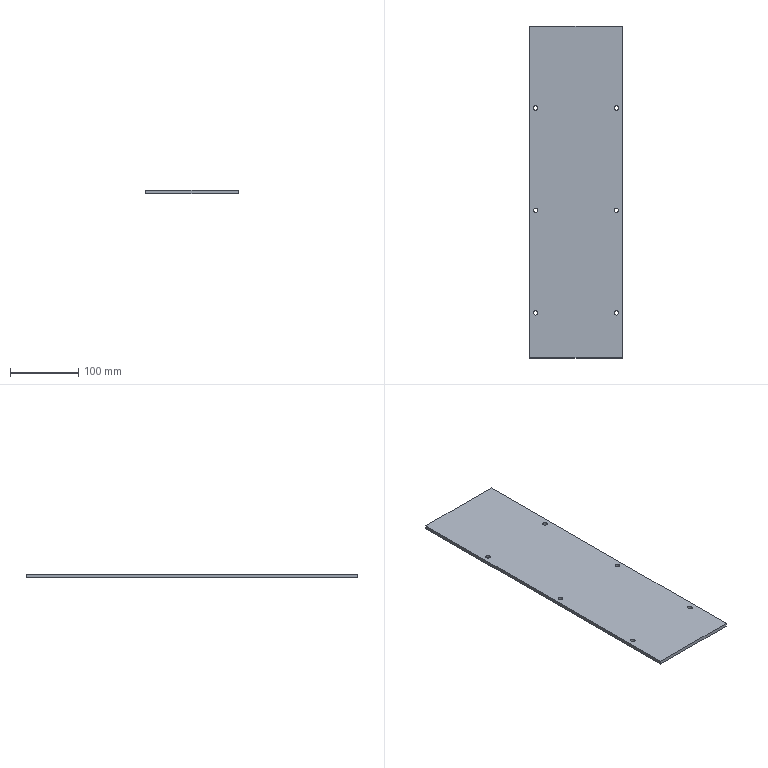Component | SolidWorks | ZL-11-03LargeUprightPlate-3 | 1 solid | 18 faces | box 136 x 486 x 5 mm | volume 329485 mm3 | cylinder 12 | plane 6 | commonest cylinder face diameters 6.5 x12
build123d program:
from build123d import *

# Parameters (mm, degrees)
SKETCH1_W                  = 136
SKETCH1_H                  = 486
EXTRUDE1_DEPTH             = 5
F_6_5_6_5_DIAMETER_HOLE1_D = 6.5
LPATTERN1_COUNT            = 2
LPATTERN1_PITCH            = 118
LPATTERN1_COUNT_DIR2       = 3
LPATTERN1_PITCH_DIR2       = 150


with BuildPart() as part:
    # Sketch1 → Extrude1 (new body)
    with BuildSketch(Plane.XY):
        Rectangle(SKETCH1_W, SKETCH1_H)
    extrude(amount=EXTRUDE1_DEPTH)

    # 6.5 _6.5_ Diameter Hole1 (through all)
    with Locations(Plane(origin=(-59, 123, 5), x_dir=(1, 0, 0), z_dir=(0, 0, 1))):
        with Locations((0, 0)):
            f_6_5_6_5_diameter_hole1 = Hole(F_6_5_6_5_DIAMETER_HOLE1_D / 2)

    # LPattern1: 6.5 _6.5_ Diameter Hole1 2 × 3
    with Locations(*[(i * LPATTERN1_PITCH, -j * LPATTERN1_PITCH_DIR2, 0) for i in range(LPATTERN1_COUNT) for j in range(LPATTERN1_COUNT_DIR2) if (i, j) != (0, 0)]):
        add(f_6_5_6_5_diameter_hole1, mode=Mode.SUBTRACT)


solid = part.part

# Placed as in the assembly
solid = solid.moved(Location((125.552, 281.22, 60.5), (0, 0, 0)))
STEP:
#1=CARTESIAN_POINT('',(7.138,4.103,2.382));
#2=VERTEX_POINT('',#1);
#3=CARTESIAN_POINT('',(7.394,4.103,2.382));
#4=VERTEX_POINT('',#3);
#5=CARTESIAN_POINT('',(7.266,4.103,2.382));
#6=DIRECTION('',(0.,0.,1.));
#7=DIRECTION('',(1.,0.,0.));
#8=AXIS2_PLACEMENT_3D('',#5,#6,#7);
#9=CIRCLE('',#8,0.128);
#10=EDGE_CURVE('',#2,#4,#9,.T.);
#11=ORIENTED_EDGE('',*,*,#10,.F.);
#12=CARTESIAN_POINT('',(7.138,4.103,2.579));
#13=VERTEX_POINT('',#12);
#14=CARTESIAN_POINT('',(7.138,4.103,2.579));
#15=DIRECTION('',(0.,0.,1.));
#16=VECTOR('',#15,39.37);
#17=LINE('',#14,#16);
#18=EDGE_CURVE('',#2,#13,#17,.T.);
#19=ORIENTED_EDGE('',*,*,#18,.T.);
#20=CARTESIAN_POINT('',(7.394,4.103,2.579));
#21=VERTEX_POINT('',#20);
#22=CARTESIAN_POINT('',(7.266,4.103,2.579));
#23=DIRECTION('',(0.,0.,1.));
#24=DIRECTION('',(1.,0.,0.));
#25=AXIS2_PLACEMENT_3D('',#22,#23,#24);
#26=CIRCLE('',#25,0.128);
#27=EDGE_CURVE('',#13,#21,#26,.T.);
#28=ORIENTED_EDGE('',*,*,#27,.T.);
#29=CARTESIAN_POINT('',(7.394,4.103,2.579));
#30=DIRECTION('',(0.,0.,1.));
#31=VECTOR('',#30,39.37);
#32=LINE('',#29,#31);
#33=EDGE_CURVE('',#4,#21,#32,.T.);
#34=ORIENTED_EDGE('',*,*,#33,.F.);
#35=EDGE_LOOP('',(#11,#19,#28,#34));
#36=FACE_OUTER_BOUND('',#35,.T.);
#37=CARTESIAN_POINT('',(7.266,4.103,2.579));
#38=DIRECTION('',(0.,0.,1.));
#39=DIRECTION('',(1.,0.,0.));
#40=AXIS2_PLACEMENT_3D('',#37,#38,#39);
#41=CYLINDRICAL_SURFACE('',#40,0.128);
#42=ADVANCED_FACE('',(#36),#41,.F.);
#43=CARTESIAN_POINT('',(7.138,10.009,2.382));
#44=VERTEX_POINT('',#43);
#45=CARTESIAN_POINT('',(7.394,10.009,2.382));
#46=VERTEX_POINT('',#45);
#47=CARTESIAN_POINT('',(7.266,10.009,2.382));
#48=DIRECTION('',(0.,0.,1.));
#49=DIRECTION('',(1.,0.,0.));
#50=AXIS2_PLACEMENT_3D('',#47,#48,#49);
#51=CIRCLE('',#50,0.128);
#52=EDGE_CURVE('',#44,#46,#51,.T.);
#53=ORIENTED_EDGE('',*,*,#52,.F.);
#54=CARTESIAN_POINT('',(7.138,10.009,2.579));
#55=VERTEX_POINT('',#54);
#56=CARTESIAN_POINT('',(7.138,10.009,2.579));
#57=DIRECTION('',(0.,0.,1.));
#58=VECTOR('',#57,39.37);
#59=LINE('',#56,#58);
#60=EDGE_CURVE('',#44,#55,#59,.T.);
#61=ORIENTED_EDGE('',*,*,#60,.T.);
#62=CARTESIAN_POINT('',(7.394,10.009,2.579));
#63=VERTEX_POINT('',#62);
#64=CARTESIAN_POINT('',(7.266,10.009,2.579));
#65=DIRECTION('',(0.,0.,1.));
#66=DIRECTION('',(1.,0.,0.));
#67=AXIS2_PLACEMENT_3D('',#64,#65,#66);
#68=CIRCLE('',#67,0.128);
#69=EDGE_CURVE('',#55,#63,#68,.T.);
#70=ORIENTED_EDGE('',*,*,#69,.T.);
#71=CARTESIAN_POINT('',(7.394,10.009,2.579));
#72=DIRECTION('',(0.,0.,1.));
#73=VECTOR('',#72,39.37);
#74=LINE('',#71,#73);
#75=EDGE_CURVE('',#46,#63,#74,.T.);
#76=ORIENTED_EDGE('',*,*,#75,.F.);
#77=EDGE_LOOP('',(#53,#61,#70,#76));
#78=FACE_OUTER_BOUND('',#77,.T.);
#79=CARTESIAN_POINT('',(7.266,10.009,2.579));
#80=DIRECTION('',(0.,0.,1.));
#81=DIRECTION('',(1.,0.,0.));
#82=AXIS2_PLACEMENT_3D('',#79,#80,#81);
#83=CYLINDRICAL_SURFACE('',#82,0.128);
#84=ADVANCED_FACE('',(#78),#83,.F.);
#85=CARTESIAN_POINT('',(7.138,15.914,2.382));
#86=VERTEX_POINT('',#85);
#87=CARTESIAN_POINT('',(7.394,15.914,2.382));
#88=VERTEX_POINT('',#87);
#89=CARTESIAN_POINT('',(7.266,15.914,2.382));
#90=DIRECTION('',(0.,0.,1.));
#91=DIRECTION('',(1.,0.,0.));
#92=AXIS2_PLACEMENT_3D('',#89,#90,#91);
#93=CIRCLE('',#92,0.128);
#94=EDGE_CURVE('',#86,#88,#93,.T.);
#95=ORIENTED_EDGE('',*,*,#94,.F.);
#96=CARTESIAN_POINT('',(7.138,15.914,2.579));
#97=VERTEX_POINT('',#96);
#98=CARTESIAN_POINT('',(7.138,15.914,2.579));
#99=DIRECTION('',(0.,0.,1.));
#100=VECTOR('',#99,39.37);
#101=LINE('',#98,#100);
#102=EDGE_CURVE('',#86,#97,#101,.T.);
#103=ORIENTED_EDGE('',*,*,#102,.T.);
#104=CARTESIAN_POINT('',(7.394,15.914,2.579));
#105=VERTEX_POINT('',#104);
#106=CARTESIAN_POINT('',(7.266,15.914,2.579));
#107=DIRECTION('',(0.,0.,1.));
#108=DIRECTION('',(1.,0.,0.));
#109=AXIS2_PLACEMENT_3D('',#106,#107,#108);
#110=CIRCLE('',#109,0.128);
#111=EDGE_CURVE('',#97,#105,#110,.T.);
#112=ORIENTED_EDGE('',*,*,#111,.T.);
#113=CARTESIAN_POINT('',(7.394,15.914,2.579));
#114=DIRECTION('',(0.,0.,1.));
#115=VECTOR('',#114,39.37);
#116=LINE('',#113,#115);
#117=EDGE_CURVE('',#88,#105,#116,.T.);
#118=ORIENTED_EDGE('',*,*,#117,.F.);
#119=EDGE_LOOP('',(#95,#103,#112,#118));
#120=FACE_OUTER_BOUND('',#119,.T.);
#121=CARTESIAN_POINT('',(7.266,15.914,2.579));
#122=DIRECTION('',(0.,0.,1.));
#123=DIRECTION('',(1.,0.,0.));
#124=AXIS2_PLACEMENT_3D('',#121,#122,#123);
#125=CYLINDRICAL_SURFACE('',#124,0.128);
#126=ADVANCED_FACE('',(#120),#125,.F.);
#127=CARTESIAN_POINT('',(2.492,4.103,2.382));
#128=VERTEX_POINT('',#127);
#129=CARTESIAN_POINT('',(2.748,4.103,2.382));
#130=VERTEX_POINT('',#129);
#131=CARTESIAN_POINT('',(2.62,4.103,2.382));
#132=DIRECTION('',(0.,0.,1.));
#133=DIRECTION('',(1.,0.,0.));
#134=AXIS2_PLACEMENT_3D('',#131,#132,#133);
#135=CIRCLE('',#134,0.128);
#136=EDGE_CURVE('',#128,#130,#135,.T.);
#137=ORIENTED_EDGE('',*,*,#136,.F.);
#138=CARTESIAN_POINT('',(2.492,4.103,2.579));
#139=VERTEX_POINT('',#138);
#140=CARTESIAN_POINT('',(2.492,4.103,2.579));
#141=DIRECTION('',(0.,0.,1.));
#142=VECTOR('',#141,39.37);
#143=LINE('',#140,#142);
#144=EDGE_CURVE('',#128,#139,#143,.T.);
#145=ORIENTED_EDGE('',*,*,#144,.T.);
#146=CARTESIAN_POINT('',(2.748,4.103,2.579));
#147=VERTEX_POINT('',#146);
#148=CARTESIAN_POINT('',(2.62,4.103,2.579));
#149=DIRECTION('',(0.,0.,1.));
#150=DIRECTION('',(1.,0.,0.));
#151=AXIS2_PLACEMENT_3D('',#148,#149,#150);
#152=CIRCLE('',#151,0.128);
#153=EDGE_CURVE('',#139,#147,#152,.T.);
#154=ORIENTED_EDGE('',*,*,#153,.T.);
#155=CARTESIAN_POINT('',(2.748,4.103,2.579));
#156=DIRECTION('',(0.,0.,1.));
#157=VECTOR('',#156,39.37);
#158=LINE('',#155,#157);
#159=EDGE_CURVE('',#130,#147,#158,.T.);
#160=ORIENTED_EDGE('',*,*,#159,.F.);
#161=EDGE_LOOP('',(#137,#145,#154,#160));
#162=FACE_OUTER_BOUND('',#161,.T.);
#163=CARTESIAN_POINT('',(2.62,4.103,2.579));
#164=DIRECTION('',(0.,0.,1.));
#165=DIRECTION('',(1.,0.,0.));
#166=AXIS2_PLACEMENT_3D('',#163,#164,#165);
#167=CYLINDRICAL_SURFACE('',#166,0.128);
#168=ADVANCED_FACE('',(#162),#167,.F.);
#169=CARTESIAN_POINT('',(2.492,10.009,2.382));
#170=VERTEX_POINT('',#169);
#171=CARTESIAN_POINT('',(2.748,10.009,2.382));
#172=VERTEX_POINT('',#171);
#173=CARTESIAN_POINT('',(2.62,10.009,2.382));
#174=DIRECTION('',(0.,0.,1.));
#175=DIRECTION('',(1.,0.,0.));
#176=AXIS2_PLACEMENT_3D('',#173,#174,#175);
#177=CIRCLE('',#176,0.128);
#178=EDGE_CURVE('',#170,#172,#177,.T.);
#179=ORIENTED_EDGE('',*,*,#178,.F.);
#180=CARTESIAN_POINT('',(2.492,10.009,2.579));
#181=VERTEX_POINT('',#180);
#182=CARTESIAN_POINT('',(2.492,10.009,2.579));
#183=DIRECTION('',(0.,0.,1.));
#184=VECTOR('',#183,39.37);
#185=LINE('',#182,#184);
#186=EDGE_CURVE('',#170,#181,#185,.T.);
#187=ORIENTED_EDGE('',*,*,#186,.T.);
#188=CARTESIAN_POINT('',(2.748,10.009,2.579));
#189=VERTEX_POINT('',#188);
#190=CARTESIAN_POINT('',(2.62,10.009,2.579));
#191=DIRECTION('',(0.,0.,1.));
#192=DIRECTION('',(1.,0.,0.));
#193=AXIS2_PLACEMENT_3D('',#190,#191,#192);
#194=CIRCLE('',#193,0.128);
#195=EDGE_CURVE('',#181,#189,#194,.T.);
#196=ORIENTED_EDGE('',*,*,#195,.T.);
#197=CARTESIAN_POINT('',(2.748,10.009,2.579));
#198=DIRECTION('',(0.,0.,1.));
#199=VECTOR('',#198,39.37);
#200=LINE('',#197,#199);
#201=EDGE_CURVE('',#172,#189,#200,.T.);
#202=ORIENTED_EDGE('',*,*,#201,.F.);
#203=EDGE_LOOP('',(#179,#187,#196,#202));
#204=FACE_OUTER_BOUND('',#203,.T.);
#205=CARTESIAN_POINT('',(2.62,10.009,2.579));
#206=DIRECTION('',(0.,0.,1.));
#207=DIRECTION('',(1.,0.,0.));
#208=AXIS2_PLACEMENT_3D('',#205,#206,#207);
#209=CYLINDRICAL_SURFACE('',#208,0.128);
#210=ADVANCED_FACE('',(#204),#209,.F.);
#211=CARTESIAN_POINT('',(2.492,15.914,2.382));
#212=VERTEX_POINT('',#211);
#213=CARTESIAN_POINT('',(2.748,15.914,2.382));
#214=VERTEX_POINT('',#213);
#215=CARTESIAN_POINT('',(2.62,15.914,2.382));
#216=DIRECTION('',(0.,0.,1.));
#217=DIRECTION('',(1.,0.,0.));
#218=AXIS2_PLACEMENT_3D('',#215,#216,#217);
#219=CIRCLE('',#218,0.128);
#220=EDGE_CURVE('',#212,#214,#219,.T.);
#221=ORIENTED_EDGE('',*,*,#220,.F.);
#222=CARTESIAN_POINT('',(2.492,15.914,2.579));
#223=VERTEX_POINT('',#222);
#224=CARTESIAN_POINT('',(2.492,15.914,2.579));
#225=DIRECTION('',(0.,0.,1.));
#226=VECTOR('',#225,39.37);
#227=LINE('',#224,#226);
#228=EDGE_CURVE('',#212,#223,#227,.T.);
#229=ORIENTED_EDGE('',*,*,#228,.T.);
#230=CARTESIAN_POINT('',(2.748,15.914,2.579));
#231=VERTEX_POINT('',#230);
#232=CARTESIAN_POINT('',(2.62,15.914,2.579));
#233=DIRECTION('',(0.,0.,1.));
#234=DIRECTION('',(1.,0.,0.));
#235=AXIS2_PLACEMENT_3D('',#232,#233,#234);
#236=CIRCLE('',#235,0.128);
#237=EDGE_CURVE('',#223,#231,#236,.T.);
#238=ORIENTED_EDGE('',*,*,#237,.T.);
#239=CARTESIAN_POINT('',(2.748,15.914,2.579));
#240=DIRECTION('',(0.,0.,1.));
#241=VECTOR('',#240,39.37);
#242=LINE('',#239,#241);
#243=EDGE_CURVE('',#214,#231,#242,.T.);
#244=ORIENTED_EDGE('',*,*,#243,.F.);
#245=EDGE_LOOP('',(#221,#229,#238,#244));
#246=FACE_OUTER_BOUND('',#245,.T.);
#247=CARTESIAN_POINT('',(2.62,15.914,2.579));
#248=DIRECTION('',(0.,0.,1.));
#249=DIRECTION('',(1.,0.,0.));
#250=AXIS2_PLACEMENT_3D('',#247,#248,#249);
#251=CYLINDRICAL_SURFACE('',#250,0.128);
#252=ADVANCED_FACE('',(#246),#251,.F.);
#253=CARTESIAN_POINT('',(2.266,20.639,2.382));
#254=VERTEX_POINT('',#253);
#255=CARTESIAN_POINT('',(2.266,1.505,2.382));
#256=VERTEX_POINT('',#255);
#257=CARTESIAN_POINT('',(2.266,20.639,2.382));
#258=DIRECTION('',(0.,-1.,0.));
#259=VECTOR('',#258,39.37);
#260=LINE('',#257,#259);
#261=EDGE_CURVE('',#254,#256,#260,.T.);
#262=ORIENTED_EDGE('',*,*,#261,.T.);
#263=CARTESIAN_POINT('',(2.266,1.505,2.579));
#264=VERTEX_POINT('',#263);
#265=CARTESIAN_POINT('',(2.266,1.505,2.579));
#266=DIRECTION('',(0.,0.,-1.));
#267=VECTOR('',#266,39.37);
#268=LINE('',#265,#267);
#269=EDGE_CURVE('',#264,#256,#268,.T.);
#270=ORIENTED_EDGE('',*,*,#269,.F.);
#271=CARTESIAN_POINT('',(2.266,20.639,2.579));
#272=VERTEX_POINT('',#271);
#273=CARTESIAN_POINT('',(2.266,20.639,2.579));
#274=DIRECTION('',(0.,-1.,0.));
#275=VECTOR('',#274,39.37);
#276=LINE('',#273,#275);
#277=EDGE_CURVE('',#272,#264,#276,.T.);
#278=ORIENTED_EDGE('',*,*,#277,.F.);
#279=CARTESIAN_POINT('',(2.266,20.639,2.579));
#280=DIRECTION('',(0.,0.,-1.));
#281=VECTOR('',#280,39.37);
#282=LINE('',#279,#281);
#283=EDGE_CURVE('',#272,#254,#282,.T.);
#284=ORIENTED_EDGE('',*,*,#283,.T.);
#285=EDGE_LOOP('',(#262,#270,#278,#284));
#286=FACE_OUTER_BOUND('',#285,.T.);
#287=CARTESIAN_POINT('',(2.266,20.639,2.579));
#288=DIRECTION('',(1.,0.,0.));
#289=DIRECTION('',(-0.,1.,0.));
#290=AXIS2_PLACEMENT_3D('',#287,#288,#289);
#291=PLANE('',#290);
#292=ADVANCED_FACE('',(#286),#291,.F.);
#293=CARTESIAN_POINT('',(7.62,1.505,2.382));
#294=VERTEX_POINT('',#293);
#295=CARTESIAN_POINT('',(2.266,1.505,2.382));
#296=DIRECTION('',(1.,0.,0.));
#297=VECTOR('',#296,39.37);
#298=LINE('',#295,#297);
#299=EDGE_CURVE('',#256,#294,#298,.T.);
#300=ORIENTED_EDGE('',*,*,#299,.T.);
#301=CARTESIAN_POINT('',(7.62,1.505,2.579));
#302=VERTEX_POINT('',#301);
#303=CARTESIAN_POINT('',(7.62,1.505,2.579));
#304=DIRECTION('',(0.,0.,-1.));
#305=VECTOR('',#304,39.37);
#306=LINE('',#303,#305);
#307=EDGE_CURVE('',#302,#294,#306,.T.);
#308=ORIENTED_EDGE('',*,*,#307,.F.);
#309=CARTESIAN_POINT('',(2.266,1.505,2.579));
#310=DIRECTION('',(1.,0.,0.));
#311=VECTOR('',#310,39.37);
#312=LINE('',#309,#311);
#313=EDGE_CURVE('',#264,#302,#312,.T.);
#314=ORIENTED_EDGE('',*,*,#313,.F.);
#315=ORIENTED_EDGE('',*,*,#269,.T.);
#316=EDGE_LOOP('',(#300,#308,#314,#315));
#317=FACE_OUTER_BOUND('',#316,.T.);
#318=CARTESIAN_POINT('',(2.266,1.505,2.579));
#319=DIRECTION('',(-0.,1.,0.));
#320=DIRECTION('',(-1.,-0.,0.));
#321=AXIS2_PLACEMENT_3D('',#318,#319,#320);
#322=PLANE('',#321);
#323=ADVANCED_FACE('',(#317),#322,.F.);
#324=CARTESIAN_POINT('',(7.62,20.639,2.382));
#325=VERTEX_POINT('',#324);
#326=CARTESIAN_POINT('',(7.62,20.639,2.382));
#327=DIRECTION('',(-0.,1.,0.));
#328=VECTOR('',#327,39.37);
#329=LINE('',#326,#328);
#330=EDGE_CURVE('',#294,#325,#329,.T.);
#331=ORIENTED_EDGE('',*,*,#330,.T.);
#332=CARTESIAN_POINT('',(7.62,20.639,2.579));
#333=VERTEX_POINT('',#332);
#334=CARTESIAN_POINT('',(7.62,20.639,2.579));
#335=DIRECTION('',(0.,0.,-1.));
#336=VECTOR('',#335,39.37);
#337=LINE('',#334,#336);
#338=EDGE_CURVE('',#333,#325,#337,.T.);
#339=ORIENTED_EDGE('',*,*,#338,.F.);
#340=CARTESIAN_POINT('',(7.62,20.639,2.579));
#341=DIRECTION('',(-0.,1.,0.));
#342=VECTOR('',#341,39.37);
#343=LINE('',#340,#342);
#344=EDGE_CURVE('',#302,#333,#343,.T.);
#345=ORIENTED_EDGE('',*,*,#344,.F.);
#346=ORIENTED_EDGE('',*,*,#307,.T.);
#347=EDGE_LOOP('',(#331,#339,#345,#346));
#348=FACE_OUTER_BOUND('',#347,.T.);
#349=CARTESIAN_POINT('',(7.62,20.639,2.579));
#350=DIRECTION('',(-1.,-0.,0.));
#351=DIRECTION('',(0.,-1.,0.));
#352=AXIS2_PLACEMENT_3D('',#349,#350,#351);
#353=PLANE('',#352);
#354=ADVANCED_FACE('',(#348),#353,.F.);
#355=CARTESIAN_POINT('',(2.266,20.639,2.382));
#356=DIRECTION('',(-1.,-0.,0.));
#357=VECTOR('',#356,39.37);
#358=LINE('',#355,#357);
#359=EDGE_CURVE('',#325,#254,#358,.T.);
#360=ORIENTED_EDGE('',*,*,#359,.T.);
#361=ORIENTED_EDGE('',*,*,#283,.F.);
#362=CARTESIAN_POINT('',(2.266,20.639,2.579));
#363=DIRECTION('',(-1.,-0.,0.));
#364=VECTOR('',#363,39.37);
#365=LINE('',#362,#364);
#366=EDGE_CURVE('',#333,#272,#365,.T.);
#367=ORIENTED_EDGE('',*,*,#366,.F.);
#368=ORIENTED_EDGE('',*,*,#338,.T.);
#369=EDGE_LOOP('',(#360,#361,#367,#368));
#370=FACE_OUTER_BOUND('',#369,.T.);
#371=CARTESIAN_POINT('',(2.266,20.639,2.579));
#372=DIRECTION('',(0.,-1.,0.));
#373=DIRECTION('',(1.,0.,0.));
#374=AXIS2_PLACEMENT_3D('',#371,#372,#373);
#375=PLANE('',#374);
#376=ADVANCED_FACE('',(#370),#375,.F.);
#377=CARTESIAN_POINT('',(7.266,4.103,2.579));
#378=DIRECTION('',(0.,0.,1.));
#379=DIRECTION('',(1.,0.,0.));
#380=AXIS2_PLACEMENT_3D('',#377,#378,#379);
#381=CIRCLE('',#380,0.128);
#382=EDGE_CURVE('',#21,#13,#381,.T.);
#383=ORIENTED_EDGE('',*,*,#382,.F.);
#384=ORIENTED_EDGE('',*,*,#27,.F.);
#385=EDGE_LOOP('',(#383,#384));
#386=FACE_BOUND('',#385,.T.);
#387=CARTESIAN_POINT('',(7.266,10.009,2.579));
#388=DIRECTION('',(0.,0.,1.));
#389=DIRECTION('',(1.,0.,0.));
#390=AXIS2_PLACEMENT_3D('',#387,#388,#389);
#391=CIRCLE('',#390,0.128);
#392=EDGE_CURVE('',#63,#55,#391,.T.);
#393=ORIENTED_EDGE('',*,*,#392,.F.);
#394=ORIENTED_EDGE('',*,*,#69,.F.);
#395=EDGE_LOOP('',(#393,#394));
#396=FACE_BOUND('',#395,.T.);
#397=CARTESIAN_POINT('',(7.266,15.914,2.579));
#398=DIRECTION('',(0.,0.,1.));
#399=DIRECTION('',(1.,0.,0.));
#400=AXIS2_PLACEMENT_3D('',#397,#398,#399);
#401=CIRCLE('',#400,0.128);
#402=EDGE_CURVE('',#105,#97,#401,.T.);
#403=ORIENTED_EDGE('',*,*,#402,.F.);
#404=ORIENTED_EDGE('',*,*,#111,.F.);
#405=EDGE_LOOP('',(#403,#404));
#406=FACE_BOUND('',#405,.T.);
#407=CARTESIAN_POINT('',(2.62,4.103,2.579));
#408=DIRECTION('',(0.,0.,1.));
#409=DIRECTION('',(1.,0.,0.));
#410=AXIS2_PLACEMENT_3D('',#407,#408,#409);
#411=CIRCLE('',#410,0.128);
#412=EDGE_CURVE('',#147,#139,#411,.T.);
#413=ORIENTED_EDGE('',*,*,#412,.F.);
#414=ORIENTED_EDGE('',*,*,#153,.F.);
#415=EDGE_LOOP('',(#413,#414));
#416=FACE_BOUND('',#415,.T.);
#417=CARTESIAN_POINT('',(2.62,10.009,2.579));
#418=DIRECTION('',(0.,0.,1.));
#419=DIRECTION('',(1.,0.,0.));
#420=AXIS2_PLACEMENT_3D('',#417,#418,#419);
#421=CIRCLE('',#420,0.128);
#422=EDGE_CURVE('',#189,#181,#421,.T.);
#423=ORIENTED_EDGE('',*,*,#422,.F.);
#424=ORIENTED_EDGE('',*,*,#195,.F.);
#425=EDGE_LOOP('',(#423,#424));
#426=FACE_BOUND('',#425,.T.);
#427=CARTESIAN_POINT('',(2.62,15.914,2.579));
#428=DIRECTION('',(0.,0.,1.));
#429=DIRECTION('',(1.,0.,0.));
#430=AXIS2_PLACEMENT_3D('',#427,#428,#429);
#431=CIRCLE('',#430,0.128);
#432=EDGE_CURVE('',#231,#223,#431,.T.);
#433=ORIENTED_EDGE('',*,*,#432,.F.);
#434=ORIENTED_EDGE('',*,*,#237,.F.);
#435=EDGE_LOOP('',(#433,#434));
#436=FACE_BOUND('',#435,.T.);
#437=ORIENTED_EDGE('',*,*,#277,.T.);
#438=ORIENTED_EDGE('',*,*,#313,.T.);
#439=ORIENTED_EDGE('',*,*,#344,.T.);
#440=ORIENTED_EDGE('',*,*,#366,.T.);
#441=EDGE_LOOP('',(#437,#438,#439,#440));
#442=FACE_OUTER_BOUND('',#441,.T.);
#443=CARTESIAN_POINT('',(2.266,20.639,2.579));
#444=DIRECTION('',(0.,0.,1.));
#445=DIRECTION('',(1.,0.,0.));
#446=AXIS2_PLACEMENT_3D('',#443,#444,#445);
#447=PLANE('',#446);
#448=ADVANCED_FACE('',(#386,#396,#406,#416,#426,#436,#442),#447,.T.);
#449=CARTESIAN_POINT('',(7.266,4.103,2.382));
#450=DIRECTION('',(0.,0.,1.));
#451=DIRECTION('',(1.,0.,0.));
#452=AXIS2_PLACEMENT_3D('',#449,#450,#451);
#453=CIRCLE('',#452,0.128);
#454=EDGE_CURVE('',#4,#2,#453,.T.);
#455=ORIENTED_EDGE('',*,*,#454,.T.);
#456=ORIENTED_EDGE('',*,*,#10,.T.);
#457=EDGE_LOOP('',(#455,#456));
#458=FACE_BOUND('',#457,.T.);
#459=CARTESIAN_POINT('',(7.266,10.009,2.382));
#460=DIRECTION('',(0.,0.,1.));
#461=DIRECTION('',(1.,0.,0.));
#462=AXIS2_PLACEMENT_3D('',#459,#460,#461);
#463=CIRCLE('',#462,0.128);
#464=EDGE_CURVE('',#46,#44,#463,.T.);
#465=ORIENTED_EDGE('',*,*,#464,.T.);
#466=ORIENTED_EDGE('',*,*,#52,.T.);
#467=EDGE_LOOP('',(#465,#466));
#468=FACE_BOUND('',#467,.T.);
#469=CARTESIAN_POINT('',(7.266,15.914,2.382));
#470=DIRECTION('',(0.,0.,1.));
#471=DIRECTION('',(1.,0.,0.));
#472=AXIS2_PLACEMENT_3D('',#469,#470,#471);
#473=CIRCLE('',#472,0.128);
#474=EDGE_CURVE('',#88,#86,#473,.T.);
#475=ORIENTED_EDGE('',*,*,#474,.T.);
#476=ORIENTED_EDGE('',*,*,#94,.T.);
#477=EDGE_LOOP('',(#475,#476));
#478=FACE_BOUND('',#477,.T.);
#479=CARTESIAN_POINT('',(2.62,4.103,2.382));
#480=DIRECTION('',(0.,0.,1.));
#481=DIRECTION('',(1.,0.,0.));
#482=AXIS2_PLACEMENT_3D('',#479,#480,#481);
#483=CIRCLE('',#482,0.128);
#484=EDGE_CURVE('',#130,#128,#483,.T.);
#485=ORIENTED_EDGE('',*,*,#484,.T.);
#486=ORIENTED_EDGE('',*,*,#136,.T.);
#487=EDGE_LOOP('',(#485,#486));
#488=FACE_BOUND('',#487,.T.);
#489=CARTESIAN_POINT('',(2.62,10.009,2.382));
#490=DIRECTION('',(0.,0.,1.));
#491=DIRECTION('',(1.,0.,0.));
#492=AXIS2_PLACEMENT_3D('',#489,#490,#491);
#493=CIRCLE('',#492,0.128);
#494=EDGE_CURVE('',#172,#170,#493,.T.);
#495=ORIENTED_EDGE('',*,*,#494,.T.);
#496=ORIENTED_EDGE('',*,*,#178,.T.);
#497=EDGE_LOOP('',(#495,#496));
#498=FACE_BOUND('',#497,.T.);
#499=CARTESIAN_POINT('',(2.62,15.914,2.382));
#500=DIRECTION('',(0.,0.,1.));
#501=DIRECTION('',(1.,0.,0.));
#502=AXIS2_PLACEMENT_3D('',#499,#500,#501);
#503=CIRCLE('',#502,0.128);
#504=EDGE_CURVE('',#214,#212,#503,.T.);
#505=ORIENTED_EDGE('',*,*,#504,.T.);
#506=ORIENTED_EDGE('',*,*,#220,.T.);
#507=EDGE_LOOP('',(#505,#506));
#508=FACE_BOUND('',#507,.T.);
#509=ORIENTED_EDGE('',*,*,#261,.F.);
#510=ORIENTED_EDGE('',*,*,#359,.F.);
#511=ORIENTED_EDGE('',*,*,#330,.F.);
#512=ORIENTED_EDGE('',*,*,#299,.F.);
#513=EDGE_LOOP('',(#509,#510,#511,#512));
#514=FACE_OUTER_BOUND('',#513,.T.);
#515=CARTESIAN_POINT('',(2.266,20.639,2.382));
#516=DIRECTION('',(0.,0.,1.));
#517=DIRECTION('',(1.,0.,0.));
#518=AXIS2_PLACEMENT_3D('',#515,#516,#517);
#519=PLANE('',#518);
#520=ADVANCED_FACE('',(#458,#468,#478,#488,#498,#508,#514),#519,.F.);
#521=ORIENTED_EDGE('',*,*,#228,.F.);
#522=ORIENTED_EDGE('',*,*,#504,.F.);
#523=ORIENTED_EDGE('',*,*,#243,.T.);
#524=ORIENTED_EDGE('',*,*,#432,.T.);
#525=EDGE_LOOP('',(#521,#522,#523,#524));
#526=FACE_OUTER_BOUND('',#525,.T.);
#527=CARTESIAN_POINT('',(2.62,15.914,2.579));
#528=DIRECTION('',(0.,0.,1.));
#529=DIRECTION('',(1.,0.,0.));
#530=AXIS2_PLACEMENT_3D('',#527,#528,#529);
#531=CYLINDRICAL_SURFACE('',#530,0.128);
#532=ADVANCED_FACE('',(#526),#531,.F.);
#533=ORIENTED_EDGE('',*,*,#186,.F.);
#534=ORIENTED_EDGE('',*,*,#494,.F.);
#535=ORIENTED_EDGE('',*,*,#201,.T.);
#536=ORIENTED_EDGE('',*,*,#422,.T.);
#537=EDGE_LOOP('',(#533,#534,#535,#536));
#538=FACE_OUTER_BOUND('',#537,.T.);
#539=CARTESIAN_POINT('',(2.62,10.009,2.579));
#540=DIRECTION('',(0.,0.,1.));
#541=DIRECTION('',(1.,0.,0.));
#542=AXIS2_PLACEMENT_3D('',#539,#540,#541);
#543=CYLINDRICAL_SURFACE('',#542,0.128);
#544=ADVANCED_FACE('',(#538),#543,.F.);
#545=ORIENTED_EDGE('',*,*,#144,.F.);
#546=ORIENTED_EDGE('',*,*,#484,.F.);
#547=ORIENTED_EDGE('',*,*,#159,.T.);
#548=ORIENTED_EDGE('',*,*,#412,.T.);
#549=EDGE_LOOP('',(#545,#546,#547,#548));
#550=FACE_OUTER_BOUND('',#549,.T.);
#551=CARTESIAN_POINT('',(2.62,4.103,2.579));
#552=DIRECTION('',(0.,0.,1.));
#553=DIRECTION('',(1.,0.,0.));
#554=AXIS2_PLACEMENT_3D('',#551,#552,#553);
#555=CYLINDRICAL_SURFACE('',#554,0.128);
#556=ADVANCED_FACE('',(#550),#555,.F.);
#557=ORIENTED_EDGE('',*,*,#102,.F.);
#558=ORIENTED_EDGE('',*,*,#474,.F.);
#559=ORIENTED_EDGE('',*,*,#117,.T.);
#560=ORIENTED_EDGE('',*,*,#402,.T.);
#561=EDGE_LOOP('',(#557,#558,#559,#560));
#562=FACE_OUTER_BOUND('',#561,.T.);
#563=CARTESIAN_POINT('',(7.266,15.914,2.579));
#564=DIRECTION('',(0.,0.,1.));
#565=DIRECTION('',(1.,0.,0.));
#566=AXIS2_PLACEMENT_3D('',#563,#564,#565);
#567=CYLINDRICAL_SURFACE('',#566,0.128);
#568=ADVANCED_FACE('',(#562),#567,.F.);
#569=ORIENTED_EDGE('',*,*,#60,.F.);
#570=ORIENTED_EDGE('',*,*,#464,.F.);
#571=ORIENTED_EDGE('',*,*,#75,.T.);
#572=ORIENTED_EDGE('',*,*,#392,.T.);
#573=EDGE_LOOP('',(#569,#570,#571,#572));
#574=FACE_OUTER_BOUND('',#573,.T.);
#575=CARTESIAN_POINT('',(7.266,10.009,2.579));
#576=DIRECTION('',(0.,0.,1.));
#577=DIRECTION('',(1.,0.,0.));
#578=AXIS2_PLACEMENT_3D('',#575,#576,#577);
#579=CYLINDRICAL_SURFACE('',#578,0.128);
#580=ADVANCED_FACE('',(#574),#579,.F.);
#581=ORIENTED_EDGE('',*,*,#18,.F.);
#582=ORIENTED_EDGE('',*,*,#454,.F.);
#583=ORIENTED_EDGE('',*,*,#33,.T.);
#584=ORIENTED_EDGE('',*,*,#382,.T.);
#585=EDGE_LOOP('',(#581,#582,#583,#584));
#586=FACE_OUTER_BOUND('',#585,.T.);
#587=CARTESIAN_POINT('',(7.266,4.103,2.579));
#588=DIRECTION('',(0.,0.,1.));
#589=DIRECTION('',(1.,0.,0.));
#590=AXIS2_PLACEMENT_3D('',#587,#588,#589);
#591=CYLINDRICAL_SURFACE('',#590,0.128);
#592=ADVANCED_FACE('',(#586),#591,.F.);
#593=CLOSED_SHELL('',(#42,#84,#126,#168,#210,#252,#292,#323,#354,#376,#448,#520,#532,#544,#556,#568,#580,#592));
#594=MANIFOLD_SOLID_BREP('',#593);
#595=CARTESIAN_POINT('',(0.,0.,0.));
#596=DIRECTION('',(0.,0.,1.));
#597=DIRECTION('',(1.,0.,0.));
#598=AXIS2_PLACEMENT_3D('',#595,#596,#597);
#599=(LENGTH_UNIT()NAMED_UNIT(*)SI_UNIT($,.METRE.));
#600=LENGTH_MEASURE_WITH_UNIT(LENGTH_MEASURE(0.0254),#599);
#601=DIMENSIONAL_EXPONENTS(1.,0.,0.,0.,0.,0.,0.);
#602=(CONVERSION_BASED_UNIT('',#600)LENGTH_UNIT()NAMED_UNIT(#601));
#603=UNCERTAINTY_MEASURE_WITH_UNIT(LENGTH_MEASURE(0.00001),#602,'','');
#604=(NAMED_UNIT(*)PLANE_ANGLE_UNIT()SI_UNIT($,.RADIAN.));
#605=(NAMED_UNIT(*)SI_UNIT($,.STERADIAN.)SOLID_ANGLE_UNIT());
#606=(GEOMETRIC_REPRESENTATION_CONTEXT(3)GLOBAL_UNCERTAINTY_ASSIGNED_CONTEXT((#603))GLOBAL_UNIT_ASSIGNED_CONTEXT((#602,#604,#605))REPRESENTATION_CONTEXT('',''));
#607=ADVANCED_BREP_SHAPE_REPRESENTATION('',(#594,#598),#606);
#608=COLOUR_RGB('',0.7922,0.8196,0.9333);
#609=FILL_AREA_STYLE_COLOUR('',#608);
#610=FILL_AREA_STYLE('',(#609));
#611=SURFACE_STYLE_FILL_AREA(#610);
#612=SURFACE_SIDE_STYLE('',(#611));
#613=SURFACE_STYLE_USAGE(.BOTH.,#612);
#614=PRESENTATION_STYLE_ASSIGNMENT((#613));
#615=STYLED_ITEM('',(#614),#594);
#616=(LENGTH_UNIT()NAMED_UNIT(*)SI_UNIT($,.METRE.));
#617=LENGTH_MEASURE_WITH_UNIT(LENGTH_MEASURE(0.0254),#616);
#618=DIMENSIONAL_EXPONENTS(1.,0.,0.,0.,0.,0.,0.);
#619=(CONVERSION_BASED_UNIT('',#617)LENGTH_UNIT()NAMED_UNIT(#618));
#620=UNCERTAINTY_MEASURE_WITH_UNIT(LENGTH_MEASURE(0.00001),#619,'','');
#621=(NAMED_UNIT(*)PLANE_ANGLE_UNIT()SI_UNIT($,.RADIAN.));
#622=(NAMED_UNIT(*)SI_UNIT($,.STERADIAN.)SOLID_ANGLE_UNIT());
#623=(GEOMETRIC_REPRESENTATION_CONTEXT(3)GLOBAL_UNCERTAINTY_ASSIGNED_CONTEXT((#620))GLOBAL_UNIT_ASSIGNED_CONTEXT((#619,#621,#622))REPRESENTATION_CONTEXT('',''));
#624=MECHANICAL_DESIGN_GEOMETRIC_PRESENTATION_REPRESENTATION('',(#615),#623);
#625=PRESENTATION_LAYER_ASSIGNMENT('','',(#615));